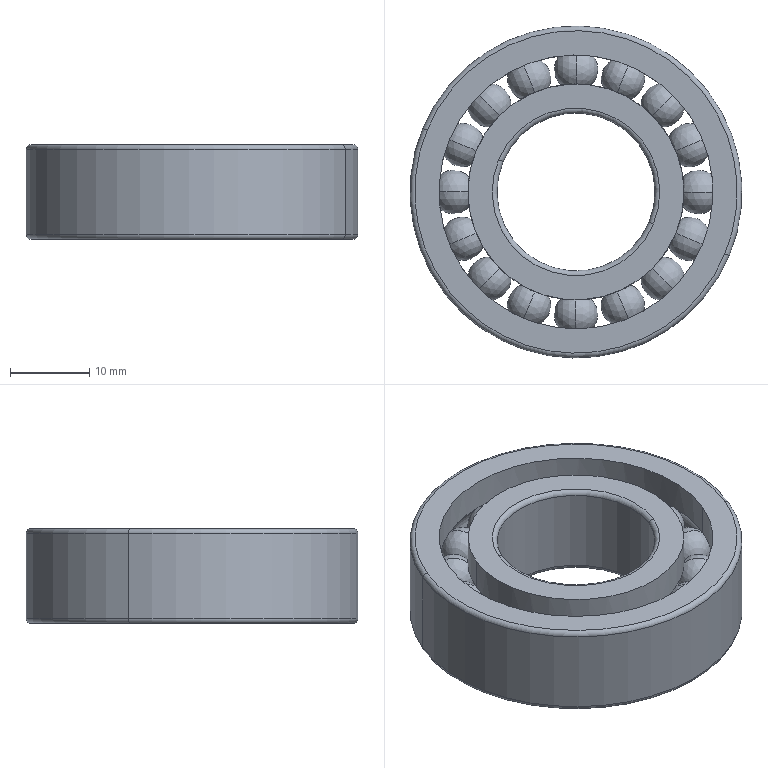Component | SolidWorks | deep groove ball bearings gb-3 | 1 solid | 104 faces | volume 9436 mm3 | torus 56 | sphere 32 | cylinder 12 | plane 4 | commonest cylinder face diameters 34.667 x4 27.333 x4 42 x2 20 x2